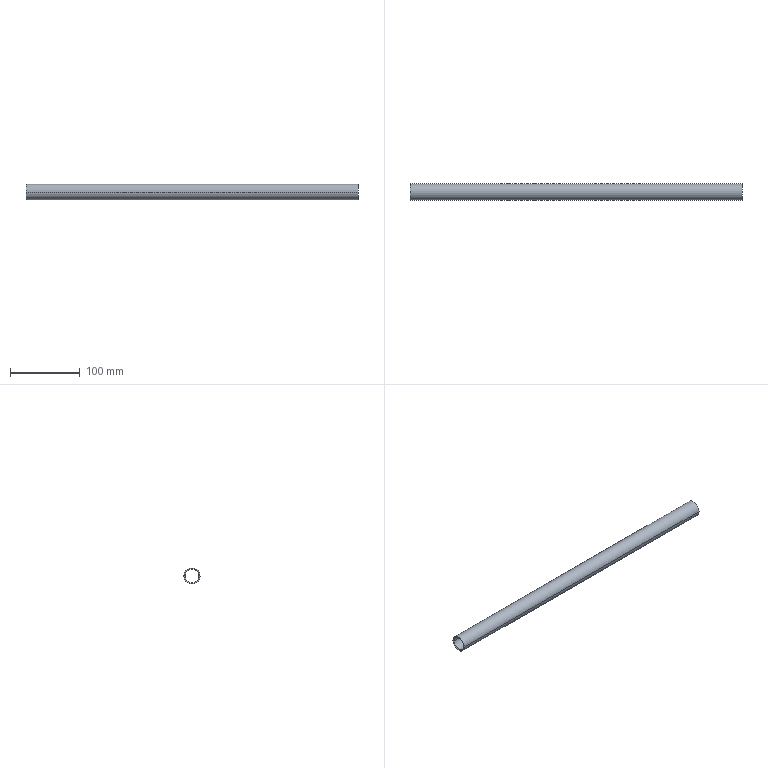Component | SolidWorks | RMS_20X400_03-1_RMS20X400_0_Barrel-1 | 1 solid | 10 faces | box 476 x 23 x 23 mm | volume 48194 mm3 | cylinder 4 | cone 4 | plane 2 | commonest cylinder face diameters 23 x2 20 x2
build123d program:
from build123d import *


with BuildPart() as part:
    # Sketch1 → Revolve1 (revolve)
    with BuildSketch(Plane.XY, mode=Mode.PRIVATE) as revolve1_sk:
        Polygon((0, 10.707), (0.7071, 10), (475.293, 10), (476, 10.707), (476, 11.5), (0, 11.5), align=None)
    revolve(revolve1_sk.sketch.rotate(Axis((476, 0, 0), (-1, 0, 0)), 270), axis=Axis((476, 0, 0), (-1, 0, 0)))


solid = part.part

# Placed as in the assembly
solid = solid.moved(Location((-12.619, 21, 41.5), (0, 0, 0)))
STEP:
#1=COLOUR_RGB('',0.7922,0.8196,0.9333);
#2=FILL_AREA_STYLE_COLOUR('',#1);
#3=FILL_AREA_STYLE('',(#2));
#4=SURFACE_STYLE_FILL_AREA(#3);
#5=SURFACE_SIDE_STYLE('',(#4));
#6=SURFACE_STYLE_USAGE(.BOTH.,#5);
#7=PRESENTATION_STYLE_ASSIGNMENT((#6));
#8=CARTESIAN_POINT('',(18.243,1.28,1.634));
#9=VERTEX_POINT('',#8);
#10=CARTESIAN_POINT('',(18.243,0.374,1.634));
#11=VERTEX_POINT('',#10);
#12=CARTESIAN_POINT('',(18.243,0.8268,1.634));
#13=DIRECTION('',(-1.,0.,0.));
#14=DIRECTION('',(0.,1.,0.));
#15=AXIS2_PLACEMENT_3D('',#12,#13,#14);
#16=CIRCLE('',#15,0.4528);
#17=EDGE_CURVE('',#9,#11,#16,.T.);
#18=ORIENTED_EDGE('',*,*,#17,.T.);
#19=CARTESIAN_POINT('',(-0.4968,0.374,1.634));
#20=VERTEX_POINT('',#19);
#21=CARTESIAN_POINT('',(18.243,0.374,1.634));
#22=DIRECTION('',(-1.,0.,0.));
#23=VECTOR('',#22,39.37);
#24=LINE('',#21,#23);
#25=EDGE_CURVE('',#11,#20,#24,.T.);
#26=ORIENTED_EDGE('',*,*,#25,.T.);
#27=CARTESIAN_POINT('',(-0.4968,1.28,1.634));
#28=VERTEX_POINT('',#27);
#29=CARTESIAN_POINT('',(-0.4968,0.8268,1.634));
#30=DIRECTION('',(-1.,0.,0.));
#31=DIRECTION('',(0.,1.,0.));
#32=AXIS2_PLACEMENT_3D('',#29,#30,#31);
#33=CIRCLE('',#32,0.4528);
#34=EDGE_CURVE('',#28,#20,#33,.T.);
#35=ORIENTED_EDGE('',*,*,#34,.F.);
#36=CARTESIAN_POINT('',(18.243,1.28,1.634));
#37=DIRECTION('',(-1.,0.,0.));
#38=VECTOR('',#37,39.37);
#39=LINE('',#36,#38);
#40=EDGE_CURVE('',#9,#28,#39,.T.);
#41=ORIENTED_EDGE('',*,*,#40,.F.);
#42=EDGE_LOOP('',(#18,#26,#35,#41));
#43=FACE_OUTER_BOUND('',#42,.T.);
#44=CARTESIAN_POINT('',(18.243,0.8268,1.634));
#45=DIRECTION('',(-1.,0.,0.));
#46=DIRECTION('',(0.,1.,0.));
#47=AXIS2_PLACEMENT_3D('',#44,#45,#46);
#48=CYLINDRICAL_SURFACE('',#47,0.4528);
#49=ADVANCED_FACE('',(#43),#48,.T.);
#50=CARTESIAN_POINT('',(18.215,0.4331,1.634));
#51=VERTEX_POINT('',#50);
#52=CARTESIAN_POINT('',(18.215,1.22,1.634));
#53=VERTEX_POINT('',#52);
#54=CARTESIAN_POINT('',(18.215,0.8268,1.634));
#55=DIRECTION('',(-1.,0.,0.));
#56=DIRECTION('',(0.,1.,0.));
#57=AXIS2_PLACEMENT_3D('',#54,#55,#56);
#58=CIRCLE('',#57,0.3937);
#59=EDGE_CURVE('',#51,#53,#58,.T.);
#60=ORIENTED_EDGE('',*,*,#59,.T.);
#61=CARTESIAN_POINT('',(18.243,1.248,1.634));
#62=VERTEX_POINT('',#61);
#63=CARTESIAN_POINT('',(18.215,1.22,1.634));
#64=DIRECTION('',(0.7071,0.7071,-0.));
#65=VECTOR('',#64,39.37);
#66=LINE('',#63,#65);
#67=EDGE_CURVE('',#53,#62,#66,.T.);
#68=ORIENTED_EDGE('',*,*,#67,.T.);
#69=CARTESIAN_POINT('',(18.243,0.4052,1.634));
#70=VERTEX_POINT('',#69);
#71=CARTESIAN_POINT('',(18.243,0.8268,1.634));
#72=DIRECTION('',(-1.,0.,0.));
#73=DIRECTION('',(0.,1.,0.));
#74=AXIS2_PLACEMENT_3D('',#71,#72,#73);
#75=CIRCLE('',#74,0.4215);
#76=EDGE_CURVE('',#70,#62,#75,.T.);
#77=ORIENTED_EDGE('',*,*,#76,.F.);
#78=CARTESIAN_POINT('',(18.215,0.4331,1.634));
#79=DIRECTION('',(0.7071,-0.7071,-0.));
#80=VECTOR('',#79,39.37);
#81=LINE('',#78,#80);
#82=EDGE_CURVE('',#51,#70,#81,.T.);
#83=ORIENTED_EDGE('',*,*,#82,.F.);
#84=EDGE_LOOP('',(#60,#68,#77,#83));
#85=FACE_OUTER_BOUND('',#84,.T.);
#86=CARTESIAN_POINT('',(18.215,0.8268,1.634));
#87=DIRECTION('',(1.,-0.,-0.));
#88=DIRECTION('',(0.,-1.,0.));
#89=AXIS2_PLACEMENT_3D('',#86,#87,#88);
#90=CONICAL_SURFACE('',#89,0.3937,0.7854);
#91=ADVANCED_FACE('',(#85),#90,.F.);
#92=ORIENTED_EDGE('',*,*,#59,.F.);
#93=CARTESIAN_POINT('',(-0.469,0.4331,1.634));
#94=VERTEX_POINT('',#93);
#95=CARTESIAN_POINT('',(18.243,0.4331,1.634));
#96=DIRECTION('',(-1.,0.,0.));
#97=VECTOR('',#96,39.37);
#98=LINE('',#95,#97);
#99=EDGE_CURVE('',#51,#94,#98,.T.);
#100=ORIENTED_EDGE('',*,*,#99,.T.);
#101=CARTESIAN_POINT('',(-0.469,1.22,1.634));
#102=VERTEX_POINT('',#101);
#103=CARTESIAN_POINT('',(-0.469,0.8268,1.634));
#104=DIRECTION('',(-1.,0.,0.));
#105=DIRECTION('',(0.,1.,0.));
#106=AXIS2_PLACEMENT_3D('',#103,#104,#105);
#107=CIRCLE('',#106,0.3937);
#108=EDGE_CURVE('',#94,#102,#107,.T.);
#109=ORIENTED_EDGE('',*,*,#108,.T.);
#110=CARTESIAN_POINT('',(18.243,1.22,1.634));
#111=DIRECTION('',(-1.,0.,0.));
#112=VECTOR('',#111,39.37);
#113=LINE('',#110,#112);
#114=EDGE_CURVE('',#53,#102,#113,.T.);
#115=ORIENTED_EDGE('',*,*,#114,.F.);
#116=EDGE_LOOP('',(#92,#100,#109,#115));
#117=FACE_OUTER_BOUND('',#116,.T.);
#118=CARTESIAN_POINT('',(18.243,0.8268,1.634));
#119=DIRECTION('',(-1.,0.,0.));
#120=DIRECTION('',(0.,1.,0.));
#121=AXIS2_PLACEMENT_3D('',#118,#119,#120);
#122=CYLINDRICAL_SURFACE('',#121,0.3937);
#123=ADVANCED_FACE('',(#117),#122,.F.);
#124=ORIENTED_EDGE('',*,*,#108,.F.);
#125=CARTESIAN_POINT('',(-0.4968,0.4052,1.634));
#126=VERTEX_POINT('',#125);
#127=CARTESIAN_POINT('',(-0.4968,0.4052,1.634));
#128=DIRECTION('',(-0.7071,-0.7071,-0.));
#129=VECTOR('',#128,39.37);
#130=LINE('',#127,#129);
#131=EDGE_CURVE('',#94,#126,#130,.T.);
#132=ORIENTED_EDGE('',*,*,#131,.T.);
#133=CARTESIAN_POINT('',(-0.4968,1.248,1.634));
#134=VERTEX_POINT('',#133);
#135=CARTESIAN_POINT('',(-0.4968,0.8268,1.634));
#136=DIRECTION('',(-1.,0.,0.));
#137=DIRECTION('',(0.,1.,0.));
#138=AXIS2_PLACEMENT_3D('',#135,#136,#137);
#139=CIRCLE('',#138,0.4215);
#140=EDGE_CURVE('',#126,#134,#139,.T.);
#141=ORIENTED_EDGE('',*,*,#140,.T.);
#142=CARTESIAN_POINT('',(-0.4968,1.248,1.634));
#143=DIRECTION('',(-0.7071,0.7071,0.));
#144=VECTOR('',#143,39.37);
#145=LINE('',#142,#144);
#146=EDGE_CURVE('',#102,#134,#145,.T.);
#147=ORIENTED_EDGE('',*,*,#146,.F.);
#148=EDGE_LOOP('',(#124,#132,#141,#147));
#149=FACE_OUTER_BOUND('',#148,.T.);
#150=CARTESIAN_POINT('',(-0.4968,0.8268,1.634));
#151=DIRECTION('',(-1.,0.,0.));
#152=DIRECTION('',(0.,1.,0.));
#153=AXIS2_PLACEMENT_3D('',#150,#151,#152);
#154=CONICAL_SURFACE('',#153,0.4215,0.7854);
#155=ADVANCED_FACE('',(#149),#154,.F.);
#156=CARTESIAN_POINT('',(-0.4968,0.8268,1.634));
#157=DIRECTION('',(-1.,0.,0.));
#158=DIRECTION('',(0.,1.,0.));
#159=AXIS2_PLACEMENT_3D('',#156,#157,#158);
#160=CIRCLE('',#159,0.4215);
#161=EDGE_CURVE('',#134,#126,#160,.T.);
#162=ORIENTED_EDGE('',*,*,#161,.F.);
#163=ORIENTED_EDGE('',*,*,#140,.F.);
#164=EDGE_LOOP('',(#162,#163));
#165=FACE_BOUND('',#164,.T.);
#166=ORIENTED_EDGE('',*,*,#34,.T.);
#167=CARTESIAN_POINT('',(-0.4968,0.8268,1.634));
#168=DIRECTION('',(-1.,0.,0.));
#169=DIRECTION('',(0.,1.,0.));
#170=AXIS2_PLACEMENT_3D('',#167,#168,#169);
#171=CIRCLE('',#170,0.4528);
#172=EDGE_CURVE('',#20,#28,#171,.T.);
#173=ORIENTED_EDGE('',*,*,#172,.T.);
#174=EDGE_LOOP('',(#166,#173));
#175=FACE_OUTER_BOUND('',#174,.T.);
#176=CARTESIAN_POINT('',(-0.4968,0.8268,1.181));
#177=DIRECTION('',(1.,-0.,-0.));
#178=DIRECTION('',(-0.,-1.,-0.));
#179=AXIS2_PLACEMENT_3D('',#176,#177,#178);
#180=PLANE('',#179);
#181=ADVANCED_FACE('',(#165,#175),#180,.F.);
#182=ORIENTED_EDGE('',*,*,#131,.F.);
#183=CARTESIAN_POINT('',(-0.469,0.8268,1.634));
#184=DIRECTION('',(-1.,0.,0.));
#185=DIRECTION('',(0.,1.,0.));
#186=AXIS2_PLACEMENT_3D('',#183,#184,#185);
#187=CIRCLE('',#186,0.3937);
#188=EDGE_CURVE('',#102,#94,#187,.T.);
#189=ORIENTED_EDGE('',*,*,#188,.F.);
#190=ORIENTED_EDGE('',*,*,#146,.T.);
#191=ORIENTED_EDGE('',*,*,#161,.T.);
#192=EDGE_LOOP('',(#182,#189,#190,#191));
#193=FACE_OUTER_BOUND('',#192,.T.);
#194=CARTESIAN_POINT('',(-0.4968,0.8268,1.634));
#195=DIRECTION('',(-1.,0.,0.));
#196=DIRECTION('',(0.,1.,0.));
#197=AXIS2_PLACEMENT_3D('',#194,#195,#196);
#198=CONICAL_SURFACE('',#197,0.4215,0.7854);
#199=ADVANCED_FACE('',(#193),#198,.F.);
#200=ORIENTED_EDGE('',*,*,#99,.F.);
#201=CARTESIAN_POINT('',(18.215,0.8268,1.634));
#202=DIRECTION('',(-1.,0.,0.));
#203=DIRECTION('',(0.,1.,0.));
#204=AXIS2_PLACEMENT_3D('',#201,#202,#203);
#205=CIRCLE('',#204,0.3937);
#206=EDGE_CURVE('',#53,#51,#205,.T.);
#207=ORIENTED_EDGE('',*,*,#206,.F.);
#208=ORIENTED_EDGE('',*,*,#114,.T.);
#209=ORIENTED_EDGE('',*,*,#188,.T.);
#210=EDGE_LOOP('',(#200,#207,#208,#209));
#211=FACE_OUTER_BOUND('',#210,.T.);
#212=CARTESIAN_POINT('',(18.243,0.8268,1.634));
#213=DIRECTION('',(-1.,0.,0.));
#214=DIRECTION('',(0.,1.,0.));
#215=AXIS2_PLACEMENT_3D('',#212,#213,#214);
#216=CYLINDRICAL_SURFACE('',#215,0.3937);
#217=ADVANCED_FACE('',(#211),#216,.F.);
#218=ORIENTED_EDGE('',*,*,#67,.F.);
#219=ORIENTED_EDGE('',*,*,#206,.T.);
#220=ORIENTED_EDGE('',*,*,#82,.T.);
#221=CARTESIAN_POINT('',(18.243,0.8268,1.634));
#222=DIRECTION('',(-1.,0.,0.));
#223=DIRECTION('',(0.,1.,0.));
#224=AXIS2_PLACEMENT_3D('',#221,#222,#223);
#225=CIRCLE('',#224,0.4215);
#226=EDGE_CURVE('',#62,#70,#225,.T.);
#227=ORIENTED_EDGE('',*,*,#226,.F.);
#228=EDGE_LOOP('',(#218,#219,#220,#227));
#229=FACE_OUTER_BOUND('',#228,.T.);
#230=CARTESIAN_POINT('',(18.215,0.8268,1.634));
#231=DIRECTION('',(1.,-0.,-0.));
#232=DIRECTION('',(0.,-1.,0.));
#233=AXIS2_PLACEMENT_3D('',#230,#231,#232);
#234=CONICAL_SURFACE('',#233,0.3937,0.7854);
#235=ADVANCED_FACE('',(#229),#234,.F.);
#236=ORIENTED_EDGE('',*,*,#17,.F.);
#237=CARTESIAN_POINT('',(18.243,0.8268,1.634));
#238=DIRECTION('',(-1.,0.,0.));
#239=DIRECTION('',(0.,1.,0.));
#240=AXIS2_PLACEMENT_3D('',#237,#238,#239);
#241=CIRCLE('',#240,0.4528);
#242=EDGE_CURVE('',#11,#9,#241,.T.);
#243=ORIENTED_EDGE('',*,*,#242,.F.);
#244=EDGE_LOOP('',(#236,#243));
#245=FACE_OUTER_BOUND('',#244,.T.);
#246=ORIENTED_EDGE('',*,*,#76,.T.);
#247=ORIENTED_EDGE('',*,*,#226,.T.);
#248=EDGE_LOOP('',(#246,#247));
#249=FACE_BOUND('',#248,.T.);
#250=CARTESIAN_POINT('',(18.243,0.8268,1.212));
#251=DIRECTION('',(-1.,0.,0.));
#252=DIRECTION('',(0.,1.,0.));
#253=AXIS2_PLACEMENT_3D('',#250,#251,#252);
#254=PLANE('',#253);
#255=ADVANCED_FACE('',(#245,#249),#254,.F.);
#256=ORIENTED_EDGE('',*,*,#25,.F.);
#257=ORIENTED_EDGE('',*,*,#242,.T.);
#258=ORIENTED_EDGE('',*,*,#40,.T.);
#259=ORIENTED_EDGE('',*,*,#172,.F.);
#260=EDGE_LOOP('',(#256,#257,#258,#259));
#261=FACE_OUTER_BOUND('',#260,.T.);
#262=CARTESIAN_POINT('',(18.243,0.8268,1.634));
#263=DIRECTION('',(-1.,0.,0.));
#264=DIRECTION('',(0.,1.,0.));
#265=AXIS2_PLACEMENT_3D('',#262,#263,#264);
#266=CYLINDRICAL_SURFACE('',#265,0.4528);
#267=ADVANCED_FACE('',(#261),#266,.T.);
#268=CLOSED_SHELL('',(#49,#91,#123,#155,#181,#199,#217,#235,#255,#267));
#269=MANIFOLD_SOLID_BREP('',#268);
#270=STYLED_ITEM('',(#7),#269);
#271=PRESENTATION_LAYER_ASSIGNMENT('','',(#270));
#272=CARTESIAN_POINT('',(0.,0.,0.));
#273=DIRECTION('',(0.,0.,1.));
#274=DIRECTION('',(1.,0.,0.));
#275=AXIS2_PLACEMENT_3D('',#272,#273,#274);
#276=(LENGTH_UNIT()NAMED_UNIT(*)SI_UNIT($,.METRE.));
#277=LENGTH_MEASURE_WITH_UNIT(LENGTH_MEASURE(0.0254),#276);
#278=DIMENSIONAL_EXPONENTS(1.,0.,0.,0.,0.,0.,0.);
#279=(CONVERSION_BASED_UNIT('',#277)LENGTH_UNIT()NAMED_UNIT(#278));
#280=UNCERTAINTY_MEASURE_WITH_UNIT(LENGTH_MEASURE(0.00001),#279,'','');
#281=(NAMED_UNIT(*)PLANE_ANGLE_UNIT()SI_UNIT($,.RADIAN.));
#282=(NAMED_UNIT(*)SI_UNIT($,.STERADIAN.)SOLID_ANGLE_UNIT());
#283=(GEOMETRIC_REPRESENTATION_CONTEXT(3)GLOBAL_UNCERTAINTY_ASSIGNED_CONTEXT((#280))GLOBAL_UNIT_ASSIGNED_CONTEXT((#279,#281,#282))REPRESENTATION_CONTEXT('',''));
#284=ADVANCED_BREP_SHAPE_REPRESENTATION('',(#269,#275),#283);
#285=(LENGTH_UNIT()NAMED_UNIT(*)SI_UNIT($,.METRE.));
#286=LENGTH_MEASURE_WITH_UNIT(LENGTH_MEASURE(0.0254),#285);
#287=DIMENSIONAL_EXPONENTS(1.,0.,0.,0.,0.,0.,0.);
#288=(CONVERSION_BASED_UNIT('',#286)LENGTH_UNIT()NAMED_UNIT(#287));
#289=UNCERTAINTY_MEASURE_WITH_UNIT(LENGTH_MEASURE(0.00001),#288,'','');
#290=(NAMED_UNIT(*)PLANE_ANGLE_UNIT()SI_UNIT($,.RADIAN.));
#291=(NAMED_UNIT(*)SI_UNIT($,.STERADIAN.)SOLID_ANGLE_UNIT());
#292=(GEOMETRIC_REPRESENTATION_CONTEXT(3)GLOBAL_UNCERTAINTY_ASSIGNED_CONTEXT((#289))GLOBAL_UNIT_ASSIGNED_CONTEXT((#288,#290,#291))REPRESENTATION_CONTEXT('',''));
#293=MECHANICAL_DESIGN_GEOMETRIC_PRESENTATION_REPRESENTATION('',(#270),#292);